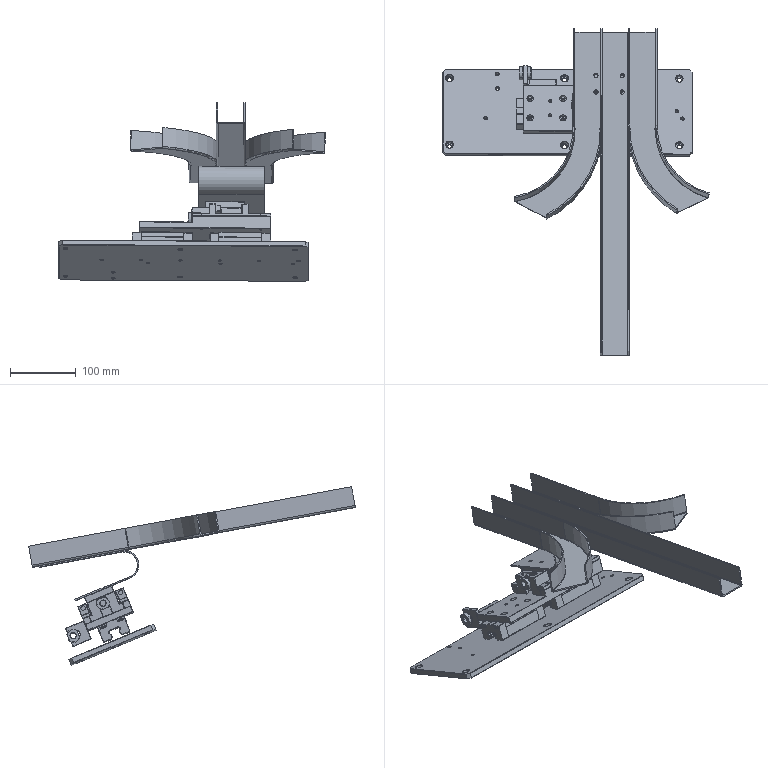Assembly | SolidWorks | mm | 13 component files | 16 solids | 1721 faces | box 405.38 x 497.67 x 272.17 mm | volume 1178421 mm3 | plane 1091 | cylinder 289 | cone 208 | spline 123 | torus 10 | commonest cylinder face diameters 6.5 x36 5 x32 1 x24 10 x20 5.5 x20 4.2 x16 2 x16 4 x14
Bill of materials:
10 | 1 |  | Rectangular block with a narrow stepped flange along each long side at the base. A transverse slot across the top splits the upper body into two raised pads. One pad has an obround through-slot reached from the side edge by a narrower open channel. The parts carry several round holes.
11 | 1 |  | Flat rectangular plate with small edge chamfers and eight holes in a symmetric layout. Two large stepped holes sit at mid-height near the left and right ends. Four medium stepped holes sit at the corners, and two smaller plain holes sit on the centreline at top and bottom.
12 | 1 |  | Long flat base plate with two raised rails along part of its length, along both long edges, so that portion has a U-shaped channel cross-section. The base has two rows of stepped holes and two small plain holes. Each rail has two small holes on its top face.
13 | 1 |  | Bracket made of a long rectangular arm joined at one end to a shorter perpendicular flange, with filleted inner corners. The arm has a long obround through-slot. Seen end-on, the flange shows a U-shaped notch open to one edge and a raised rectangular pad with relief grooves.
14 | 1 |  | Long narrow rectangular bar with two square upright blocks rising from it, spaced inboard of the ends. Each block has a round through-bore across it. The bar has a stepped hole near each end.
15 | 1 |  | Thin-walled, sheet-like trough assembly. A straight U-channel runs the full length, and two curved U-channel branches sweep outward to either side, giving a branching or junction outline in plan view. A bent strip with four small holes is near the junction. A thin curved hook-like element shows in the side view.
16 | 1 |  | Simple rectangular bar with chamfered edges and two stepped holes through its broad face.
CylinderConnector | 2 |  | Long narrow rectangular bar with two square upright blocks rising from it, spaced inboard of the ends. Each block has a round through-bore across it. The bar has a stepped hole near each end.
Mirror_A026174z0-123 | 1 |  | Spool-shaped round part: two equal end flanges joined by a smaller-diameter neck, with a plain central through-bore. Each flange is round with two parallel flats and chamfered edges.
MQBHGH20H174z0-123 | 2 |  | Rectangular block with a longitudinal channel open on the underside. The channel walls have rounded side grooves along their length. The top face has four holes and shallow lengthwise grooves, and the end sections have a slightly different outline from the central body.
NestingBasePlate | 1 |  | Long thin rectangular plate with chamfered corners. Six stepped holes sit at the corners and at the middle of each long edge, and smaller plain holes are scattered across the face.
Mates:
1. coincident | 10-1 face at (94.012, -68.436, 468.572) dir (0.006385, 0.3824, 0.924) | 11-1 face at (104.012, -68.459, 468.513) dir (-0.006385, -0.3824, -0.924)
2. coincident | 10-1 face at (134.007, -43.119, 457.818) dir (1, -0.002314, -0.005953) | 11-1 face at (134.072, -43.915, 468.97) dir (1, -0.002314, -0.005953)
3. distance | 11-1 face at (134.072, -43.915, 468.97) dir (-0.0001384, 0.924, -0.3824) | 10-1 face at (134.007, -43.119, 457.818) dir (-0.0001384, 0.924, -0.3824)
4. coincident | 10-1 face at (93.82, -79.908, 440.853) dir (-0.006385, -0.3824, -0.924) | 12-1 face at (173.823, -105.503, 450.894) dir (0.006385, 0.3824, 0.924)
5. coincident | 10-1 face at (134.015, -93.938, 478.851) dir (0.0001384, -0.924, 0.3824) | 12-1 face at (173.823, -105.503, 450.894) dir (-0.0001384, 0.924, -0.3824)
6. parallel | 10-1 face at (94.012, -68.436, 468.572) dir (0.006385, 0.3824, 0.924) | CylinderConnector-1 face at (48.004, -73.771, 469.475) dir (0.006385, 0.3824, 0.924)
7. coincident | 10-1 face at (54.009, -42.934, 458.294) dir (-1, 0.002314, 0.005953) | 12-1 face at (53.816, -45.166, 426.751) dir (-1, 0.002314, 0.005953)
8. coincident | 10-1 face at (54.009, -42.934, 458.294) dir (-1, 0.002314, 0.005953) | CylinderConnector-1 face at (53.949, -72.168, 459.571) dir (1, -0.002314, -0.005953)
9. coincident | 12-1 face at (73.757, -83.686, 431.733) dir (-0.006385, -0.3824, -0.924) | MQBHGH20HA-1/MQBHGH20H174z0-123-2 face at (160.258, -103.29, 439.248) dir (0.006385, 0.3824, 0.924)
10. coincident | 12-1 face at (173.75, -49.268, 416.797) dir (-0.0001384, 0.924, -0.3824) | 13-1 face at (23.855, -42.802, 432.473) dir (0.0001384, -0.924, 0.3824)
11. coincident | 12-1 face at (-26.236, -118.104, 446.669) dir (-1, 0.002314, 0.005953) | 13-1 face at (-26.148, -14.967, 421.298) dir (-1, 0.002314, 0.005953)
12. coincident | CylinderConnector-2 face at (-20.243, -26.723, 409.889) dir (-1, 0.002314, 0.005953) | 13-1 face at (-20.337, -44.933, 401.192) dir (1, -0.002314, -0.005953)
13. distance | CylinderConnector-2 face at (-32.775, -36.562, 408.346) dir (0.0001384, -0.924, 0.3824) | 13-1 face at (-1.337, -44.977, 401.079) dir (-0.0001384, 0.924, -0.3824)
14. coincident | 12-1 face at (173.823, -105.503, 450.894) dir (0.006385, 0.3824, 0.924) | 13-1 face at (23.817, -45.097, 426.929) dir (0.006385, 0.3824, 0.924)
15. coincident | 12-1 face at (73.885, -76.038, 450.212) dir (0.006385, 0.3824, 0.924) | 14-1 face at (113.88, -47.487, 438.119) dir (-0.006385, -0.3824, -0.924)
16. coincident | 12-1 face at (173.75, -49.268, 416.797) dir (-0.0001384, 0.924, -0.3824) | 14-1 face at (53.88, -41.342, 435.99) dir (-0.0001384, 0.924, -0.3824)
17. coincident | 12-1 face at (53.816, -45.166, 426.751) dir (-1, 0.002314, 0.005953) | 14-1 face at (53.88, -41.342, 435.99) dir (-1, 0.002314, 0.005953)
18. coincident | 12-1 face at (173.76, -118.567, 445.478) dir (1, -0.002314, -0.005953) | MQBHGH20HA-1/MQBHGH20H174z0-123-2 face at (173.675, -88.698, 419.588) dir (1, -0.002314, -0.005953)
19. width | MQBHGH20HA-1/MQBHGH20H174z0-123-2 face at (160.246, -63.941, 421.881) dir (-0.0001384, 0.924, -0.3824) | MQBHGH20HA-1/MQBHGH20H174z0-123-2 face at (160.207, -107.273, 432.239) dir (0.0001384, -0.924, 0.3824) | 12-1 face at (173.76, -118.567, 445.478) dir (0.0001384, -0.924, 0.3824) | 12-1 face at (173.75, -49.268, 416.797) dir (-0.0001384, 0.924, -0.3824)
20. coincident | 11-1 face at (104.076, -64.635, 477.753) dir (0.006385, 0.3824, 0.924) | 15-1 face at (113.121, -370.834, 604.419) dir (-0.006385, -0.3824, -0.924)
21. coincident | assembly face at (381.358, -86.631, 398.357) dir (-0.006385, -0.3824, -0.924) | NestingBasePlate-1 face at (41.365, -84.92, 399.999) dir (0.006385, 0.3824, 0.924)
22. coincident | assembly face at (231.361, -86.284, 399.25) dir (1, -0.002314, -0.005953) | NestingBasePlate-1 face at (231.37, -150.039, 425.637) dir (1, -0.002314, -0.005953)
23. coincident | 10-1 face at (97.93, -36.075, 442.164) dir (-1, 0.002314, 0.005953) | 16-1 face at (98.004, -103.86, 481.041) dir (1, -0.002314, -0.005953)
24. coincident | 10-1 edge at (89.932, -52.688, 449.095) dir (0.0001384, -0.924, 0.3824) | 16-1 face at (89.941, -107.665, 471.849) dir (-0.006385, -0.3824, -0.924)
25. coincident | 14-1 face at (53.88, -41.342, 435.99) dir (-0.0001384, 0.924, -0.3824) | 16-1 face at (93.962, -36.463, 447.764) dir (-0.0001384, 0.924, -0.3824)
26. distance | 15-1 face at (164.069, -30.124, 463.055) dir (-0.0001384, 0.924, -0.3824) | 11-1 face at (134.072, -43.915, 468.97) dir (-0.0001384, 0.924, -0.3824)
27. distance | 15-1 face at (64.071, -29.893, 463.65) dir (-1, 0.002314, 0.005953) | 11-1 face at (74.073, -43.776, 469.327) dir (-1, 0.002314, 0.005953)
28. coincident | MQBHGH20H174z0-123-1 face at (31.708, 13.457, -69.449) dir (0, 1, 0) | MQBHGH20H174z0-123-2 face at (31.708, 13.457, -188.049) dir (0, 1, 0)
29. coincident | MQBHGH20H174z0-123-1 face at (21.708, 12.457, -69.449) dir (-1, 0, 0) | MQBHGH20H174z0-123-2 face at (21.708, 12.457, -188.049) dir (-1, 0, 0)